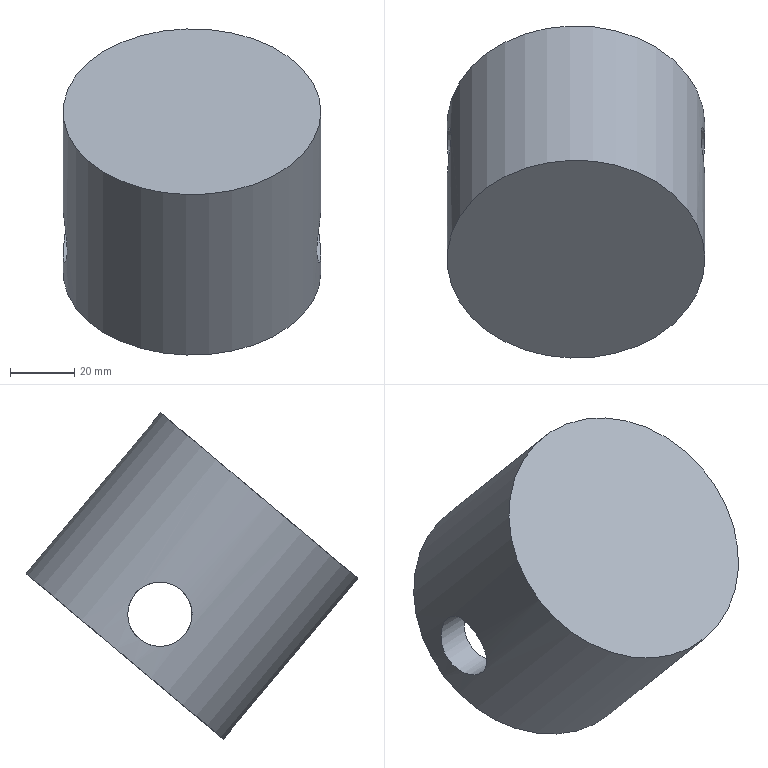Component | NX | PISTON | 1 solid | 18 faces | volume 234437 mm3 | cylinder 9 | plane 9 | commonest cylinder face diameters 60 x4 20 x4 80 x1